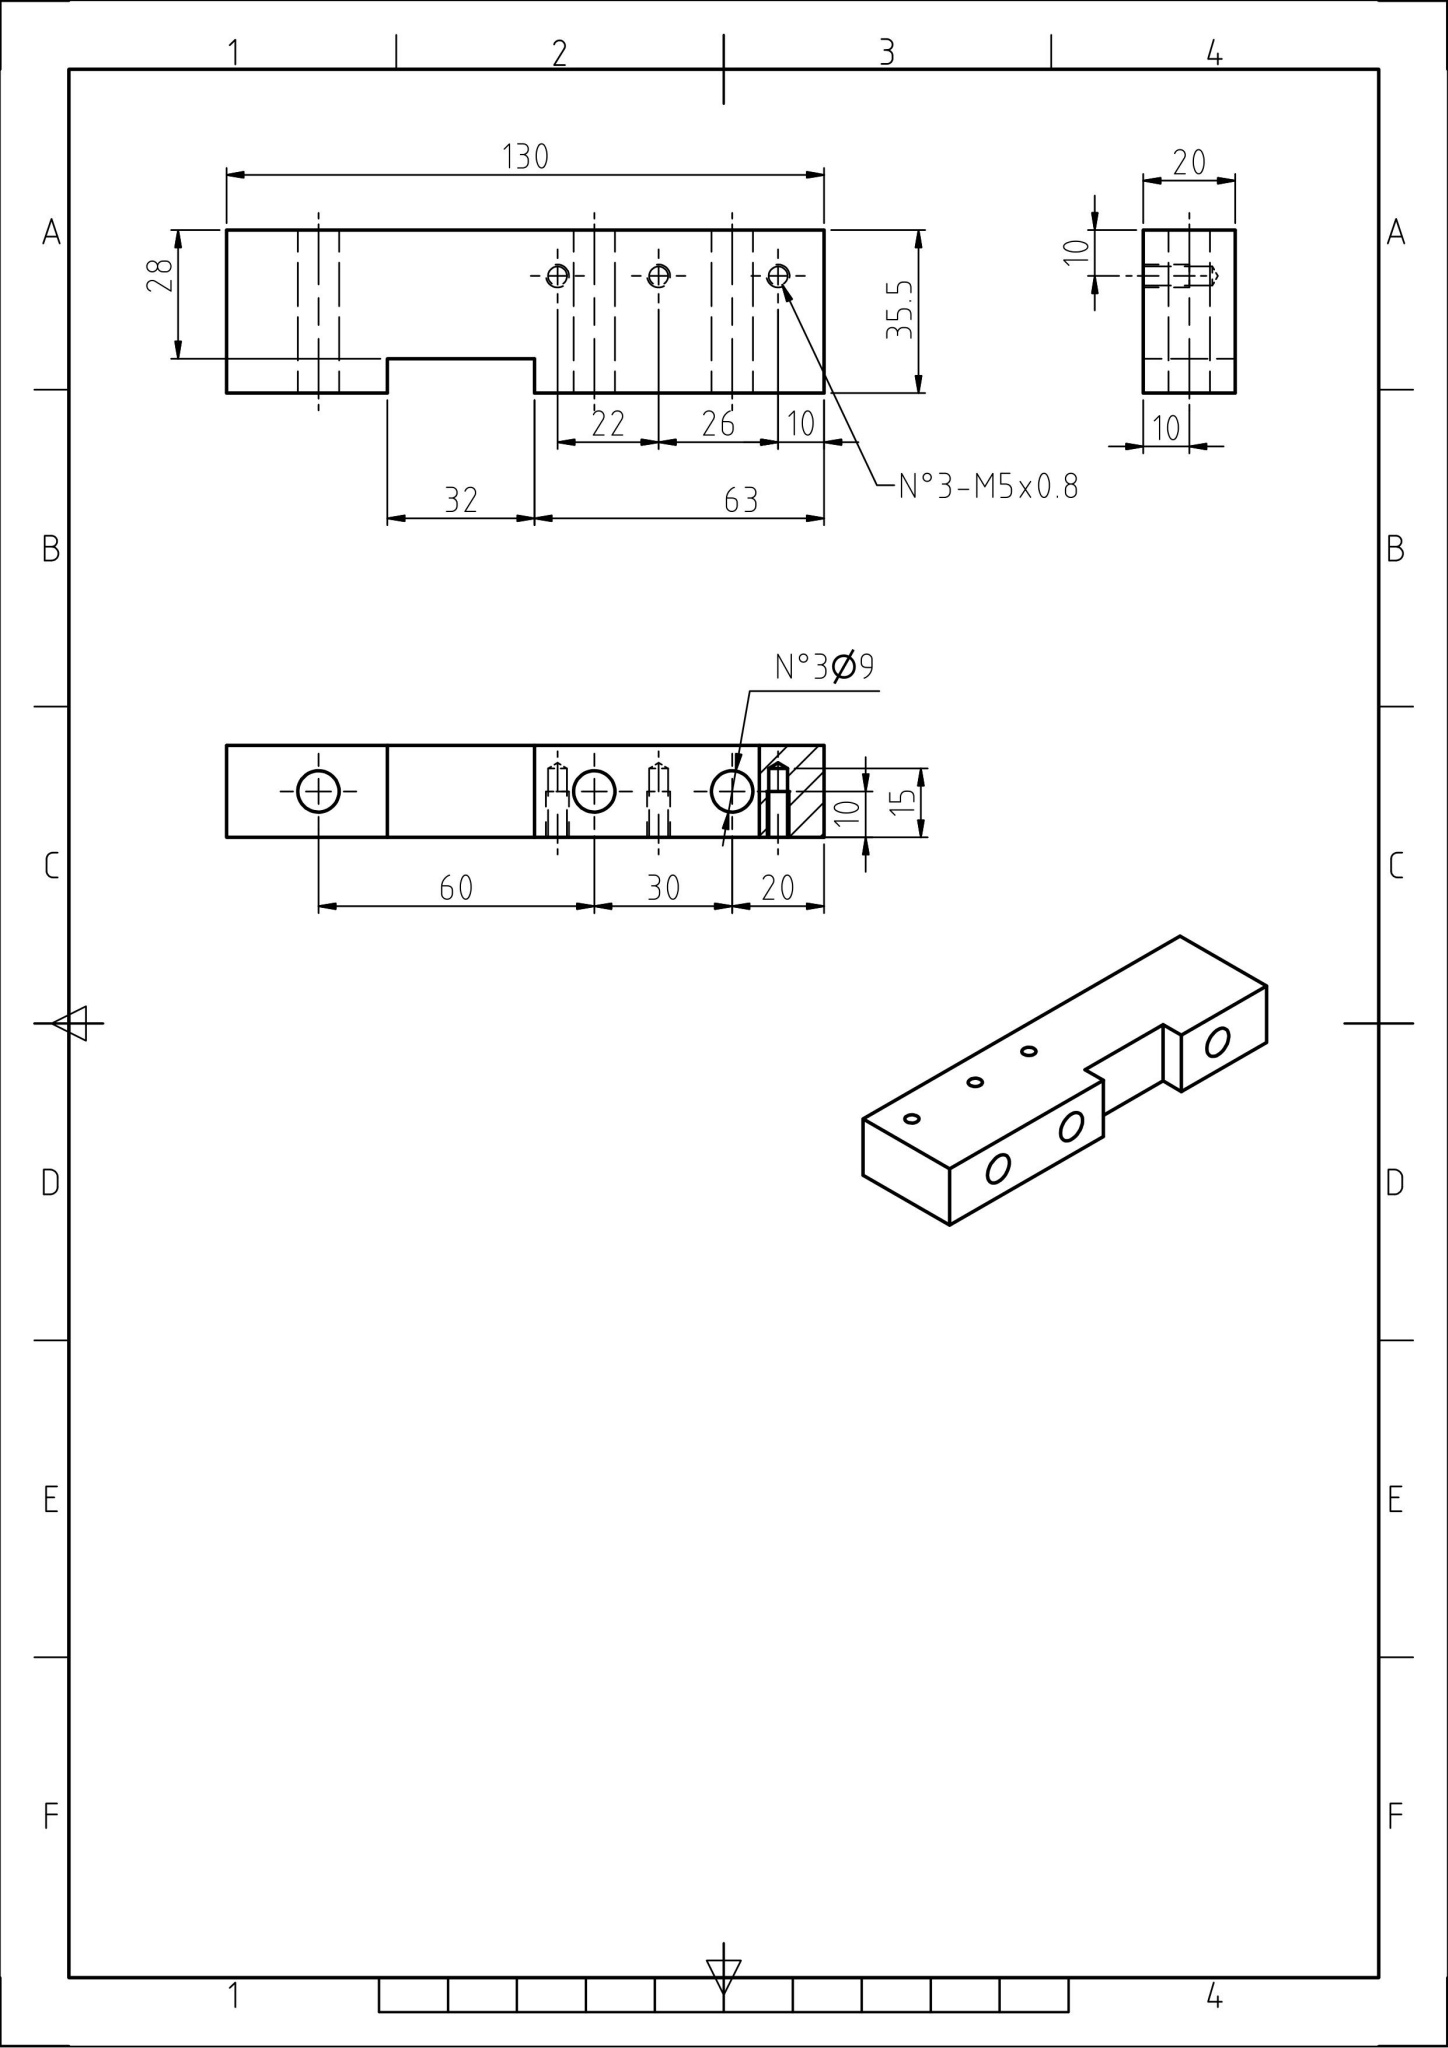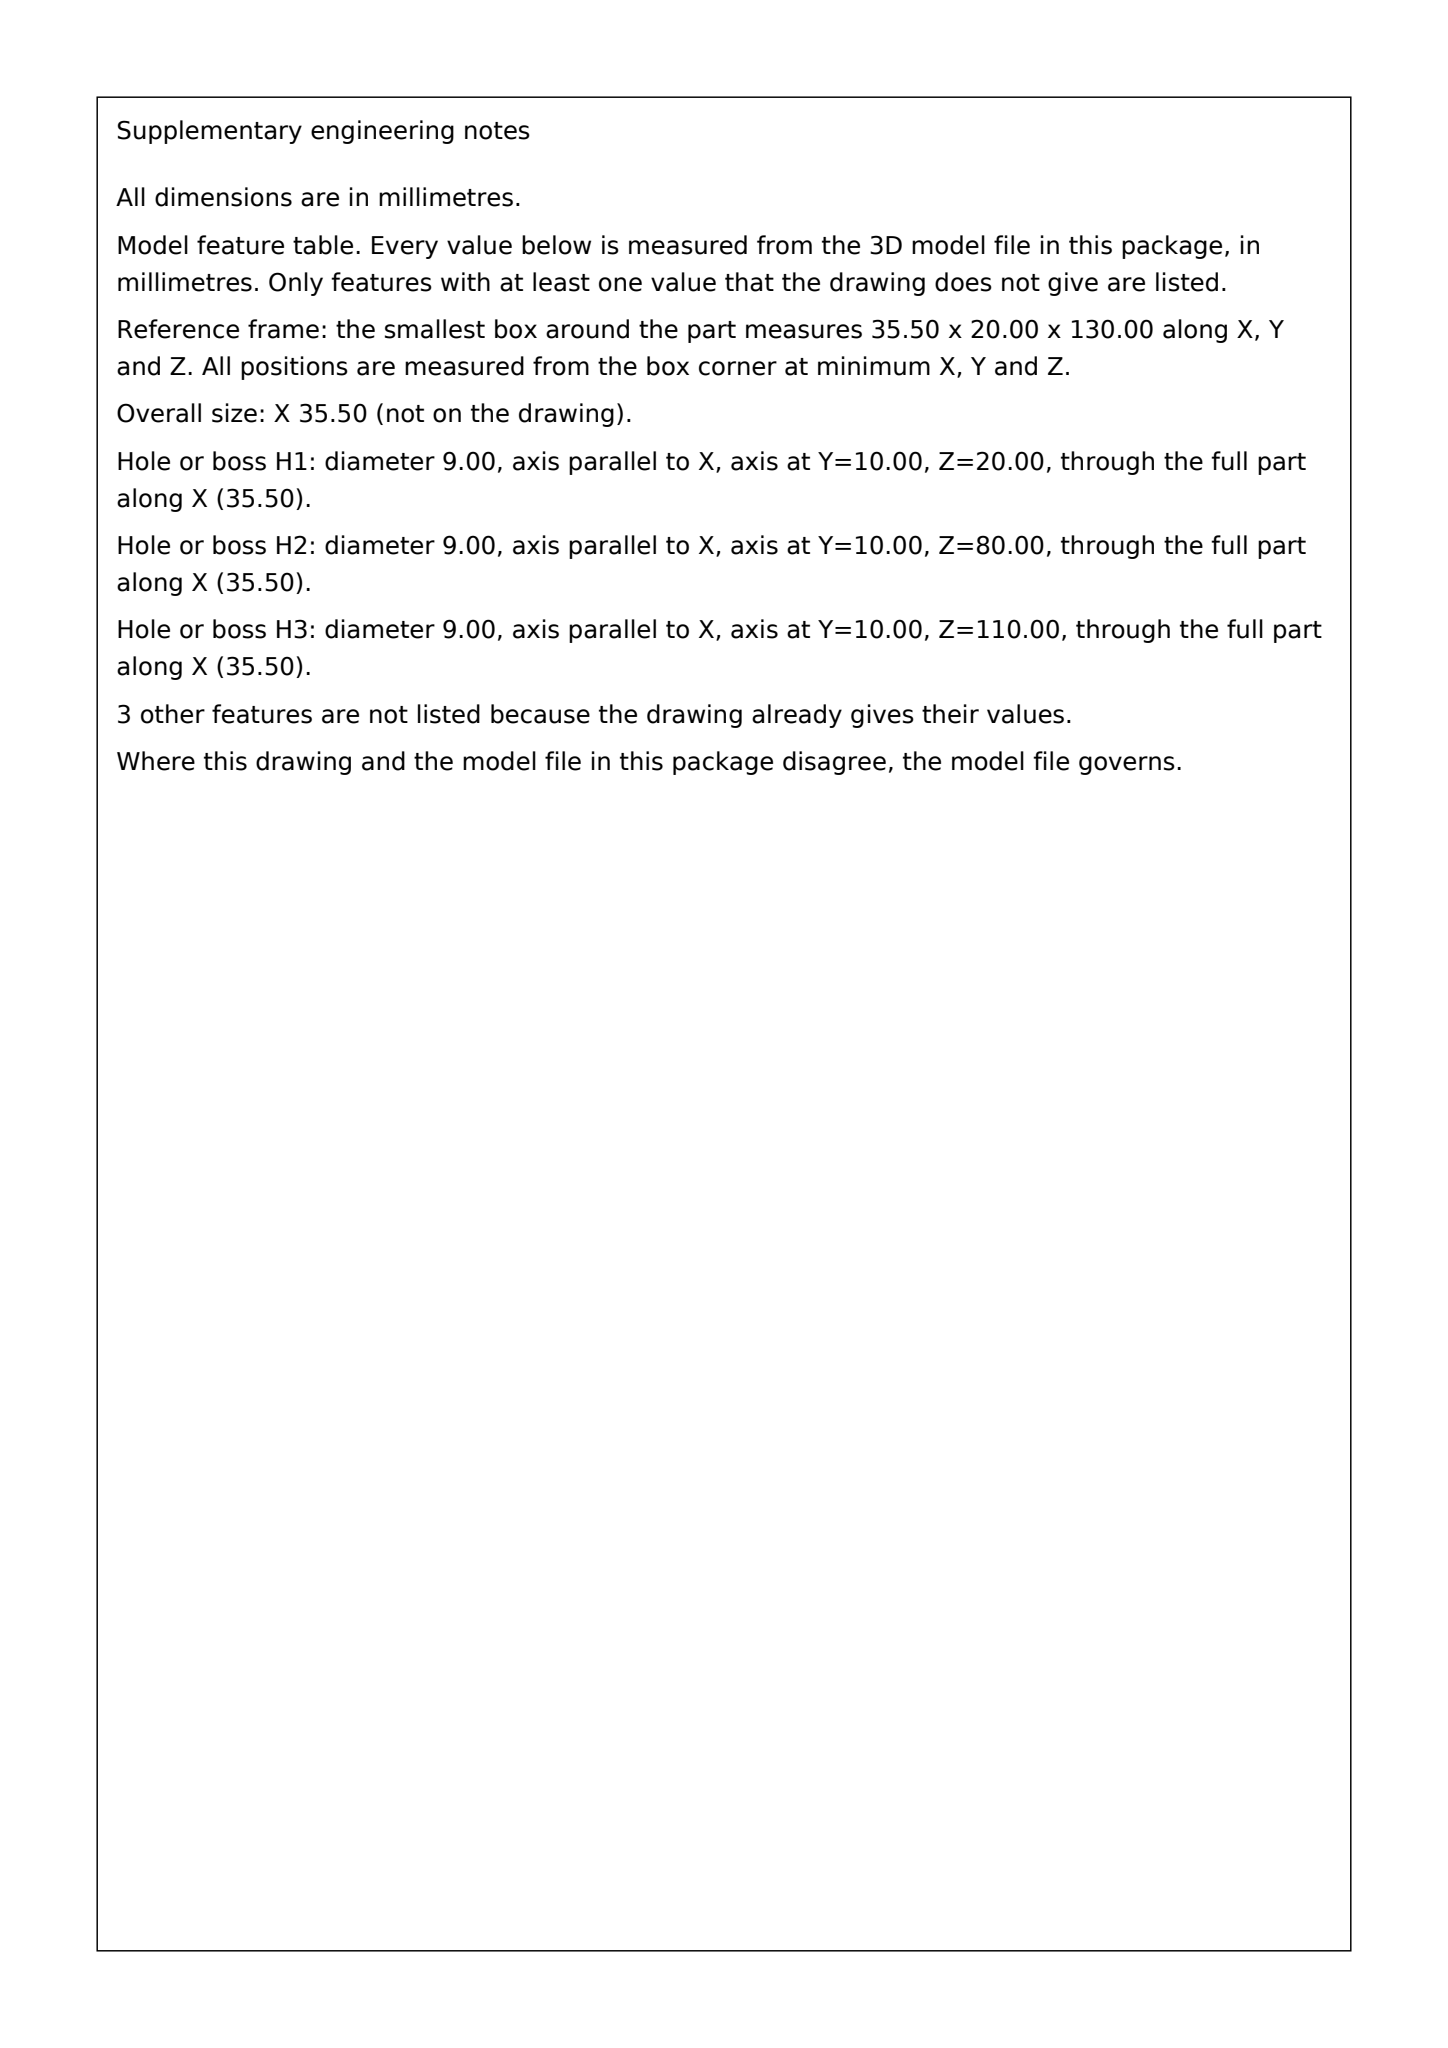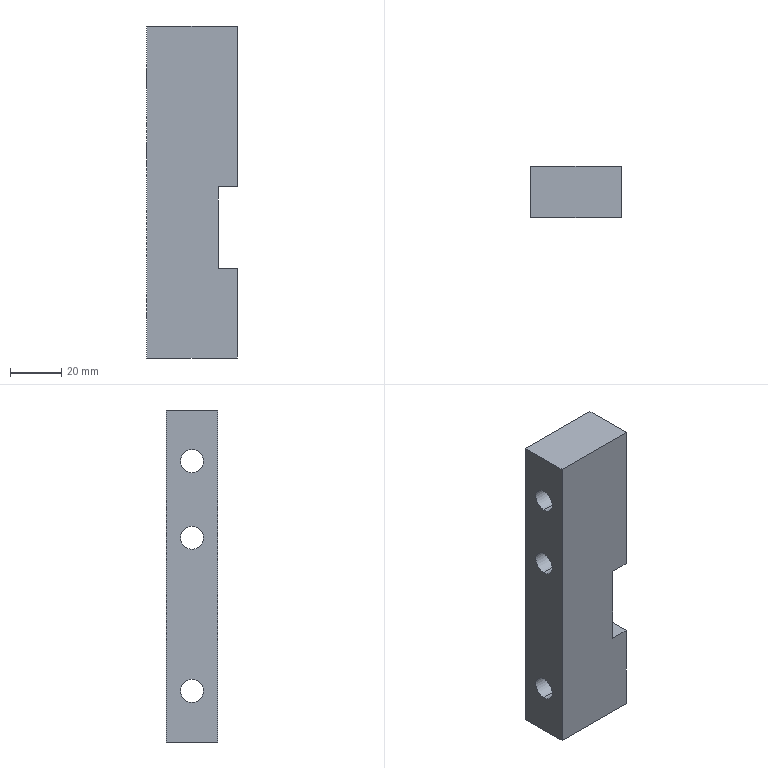Part | SolidWorks | mm | 1 solid | 28 faces | box 35.5 x 20 x 130 mm | volume 80104 mm3 | cylinder 12 | plane 10 | cone 6 | commonest cylinder face diameters 9 x6 4.134 x6
STEP:
#1=CARTESIAN_POINT('',(0.,0.,-40.5));
#2=VERTEX_POINT('',#1);
#3=CARTESIAN_POINT('',(0.,0.,-49.5));
#4=VERTEX_POINT('',#3);
#5=CARTESIAN_POINT('',(0.,0.,-45.));
#6=DIRECTION('',(1.,0.,0.));
#7=DIRECTION('',(0.,0.,-1.));
#8=AXIS2_PLACEMENT_3D('',#5,#6,#7);
#9=CIRCLE('',#8,4.5);
#10=EDGE_CURVE('',#2,#4,#9,.T.);
#11=ORIENTED_EDGE('',*,*,#10,.F.);
#12=CARTESIAN_POINT('',(35.5,0.,-40.5));
#13=VERTEX_POINT('',#12);
#14=CARTESIAN_POINT('',(-100.736,0.,-40.5));
#15=DIRECTION('',(1.,0.,0.));
#16=VECTOR('',#15,1000.);
#17=LINE('',#14,#16);
#18=EDGE_CURVE('',#2,#13,#17,.T.);
#19=ORIENTED_EDGE('',*,*,#18,.T.);
#20=CARTESIAN_POINT('',(35.5,0.,-49.5));
#21=VERTEX_POINT('',#20);
#22=CARTESIAN_POINT('',(35.5,0.,-45.));
#23=DIRECTION('',(-1.,0.,0.));
#24=DIRECTION('',(0.,0.,-1.));
#25=AXIS2_PLACEMENT_3D('',#22,#23,#24);
#26=CIRCLE('',#25,4.5);
#27=EDGE_CURVE('',#21,#13,#26,.T.);
#28=ORIENTED_EDGE('',*,*,#27,.F.);
#29=CARTESIAN_POINT('',(-100.736,0.,-49.5));
#30=DIRECTION('',(1.,0.,0.));
#31=VECTOR('',#30,1000.);
#32=LINE('',#29,#31);
#33=EDGE_CURVE('',#4,#21,#32,.T.);
#34=ORIENTED_EDGE('',*,*,#33,.F.);
#35=EDGE_LOOP('',(#11,#19,#28,#34));
#36=FACE_OUTER_BOUND('',#35,.T.);
#37=CARTESIAN_POINT('',(-100.736,0.,-45.));
#38=DIRECTION('',(1.,0.,0.));
#39=DIRECTION('',(0.,0.,-1.));
#40=AXIS2_PLACEMENT_3D('',#37,#38,#39);
#41=CYLINDRICAL_SURFACE('',#40,4.5);
#42=ADVANCED_FACE('',(#36),#41,.F.);
#43=CARTESIAN_POINT('',(0.,0.,49.5));
#44=VERTEX_POINT('',#43);
#45=CARTESIAN_POINT('',(0.,0.,40.5));
#46=VERTEX_POINT('',#45);
#47=CARTESIAN_POINT('',(0.,0.,45.));
#48=DIRECTION('',(1.,0.,0.));
#49=DIRECTION('',(0.,0.,-1.));
#50=AXIS2_PLACEMENT_3D('',#47,#48,#49);
#51=CIRCLE('',#50,4.5);
#52=EDGE_CURVE('',#44,#46,#51,.T.);
#53=ORIENTED_EDGE('',*,*,#52,.F.);
#54=CARTESIAN_POINT('',(35.5,0.,49.5));
#55=VERTEX_POINT('',#54);
#56=CARTESIAN_POINT('',(-100.736,0.,49.5));
#57=DIRECTION('',(1.,0.,0.));
#58=VECTOR('',#57,1000.);
#59=LINE('',#56,#58);
#60=EDGE_CURVE('',#44,#55,#59,.T.);
#61=ORIENTED_EDGE('',*,*,#60,.T.);
#62=CARTESIAN_POINT('',(35.5,0.,40.5));
#63=VERTEX_POINT('',#62);
#64=CARTESIAN_POINT('',(35.5,0.,45.));
#65=DIRECTION('',(-1.,0.,0.));
#66=DIRECTION('',(0.,0.,-1.));
#67=AXIS2_PLACEMENT_3D('',#64,#65,#66);
#68=CIRCLE('',#67,4.5);
#69=EDGE_CURVE('',#63,#55,#68,.T.);
#70=ORIENTED_EDGE('',*,*,#69,.F.);
#71=CARTESIAN_POINT('',(-100.736,0.,40.5));
#72=DIRECTION('',(1.,0.,0.));
#73=VECTOR('',#72,1000.);
#74=LINE('',#71,#73);
#75=EDGE_CURVE('',#46,#63,#74,.T.);
#76=ORIENTED_EDGE('',*,*,#75,.F.);
#77=EDGE_LOOP('',(#53,#61,#70,#76));
#78=FACE_OUTER_BOUND('',#77,.T.);
#79=CARTESIAN_POINT('',(-100.736,0.,45.));
#80=DIRECTION('',(1.,0.,0.));
#81=DIRECTION('',(0.,0.,-1.));
#82=AXIS2_PLACEMENT_3D('',#79,#80,#81);
#83=CYLINDRICAL_SURFACE('',#82,4.5);
#84=ADVANCED_FACE('',(#78),#83,.F.);
#85=CARTESIAN_POINT('',(0.,0.,19.5));
#86=VERTEX_POINT('',#85);
#87=CARTESIAN_POINT('',(0.,0.,10.5));
#88=VERTEX_POINT('',#87);
#89=CARTESIAN_POINT('',(0.,0.,15.));
#90=DIRECTION('',(1.,0.,0.));
#91=DIRECTION('',(0.,0.,-1.));
#92=AXIS2_PLACEMENT_3D('',#89,#90,#91);
#93=CIRCLE('',#92,4.5);
#94=EDGE_CURVE('',#86,#88,#93,.T.);
#95=ORIENTED_EDGE('',*,*,#94,.F.);
#96=CARTESIAN_POINT('',(35.5,0.,19.5));
#97=VERTEX_POINT('',#96);
#98=CARTESIAN_POINT('',(-100.736,0.,19.5));
#99=DIRECTION('',(1.,0.,0.));
#100=VECTOR('',#99,1000.);
#101=LINE('',#98,#100);
#102=EDGE_CURVE('',#86,#97,#101,.T.);
#103=ORIENTED_EDGE('',*,*,#102,.T.);
#104=CARTESIAN_POINT('',(35.5,0.,10.5));
#105=VERTEX_POINT('',#104);
#106=CARTESIAN_POINT('',(35.5,0.,15.));
#107=DIRECTION('',(-1.,0.,0.));
#108=DIRECTION('',(0.,0.,-1.));
#109=AXIS2_PLACEMENT_3D('',#106,#107,#108);
#110=CIRCLE('',#109,4.5);
#111=EDGE_CURVE('',#105,#97,#110,.T.);
#112=ORIENTED_EDGE('',*,*,#111,.F.);
#113=CARTESIAN_POINT('',(-100.736,0.,10.5));
#114=DIRECTION('',(1.,0.,0.));
#115=VECTOR('',#114,1000.);
#116=LINE('',#113,#115);
#117=EDGE_CURVE('',#88,#105,#116,.T.);
#118=ORIENTED_EDGE('',*,*,#117,.F.);
#119=EDGE_LOOP('',(#95,#103,#112,#118));
#120=FACE_OUTER_BOUND('',#119,.T.);
#121=CARTESIAN_POINT('',(-100.736,0.,15.));
#122=DIRECTION('',(1.,0.,0.));
#123=DIRECTION('',(0.,0.,-1.));
#124=AXIS2_PLACEMENT_3D('',#121,#122,#123);
#125=CYLINDRICAL_SURFACE('',#124,4.5);
#126=ADVANCED_FACE('',(#120),#125,.F.);
#127=CARTESIAN_POINT('',(7.933,-5.,7.));
#128=VERTEX_POINT('',#127);
#129=CARTESIAN_POINT('',(12.067,-5.,7.));
#130=VERTEX_POINT('',#129);
#131=CARTESIAN_POINT('',(10.,-5.,7.));
#132=DIRECTION('',(0.,1.,-0.));
#133=DIRECTION('',(1.,0.,0.));
#134=AXIS2_PLACEMENT_3D('',#131,#132,#133);
#135=CIRCLE('',#134,2.067);
#136=EDGE_CURVE('',#128,#130,#135,.T.);
#137=ORIENTED_EDGE('',*,*,#136,.F.);
#138=CARTESIAN_POINT('',(7.933,10.,7.));
#139=VERTEX_POINT('',#138);
#140=CARTESIAN_POINT('',(7.933,2.5,7.));
#141=DIRECTION('',(0.,1.,-0.));
#142=VECTOR('',#141,1000.);
#143=LINE('',#140,#142);
#144=EDGE_CURVE('',#128,#139,#143,.T.);
#145=ORIENTED_EDGE('',*,*,#144,.T.);
#146=CARTESIAN_POINT('',(12.067,10.,7.));
#147=VERTEX_POINT('',#146);
#148=CARTESIAN_POINT('',(10.,10.,7.));
#149=DIRECTION('',(0.,-1.,0.));
#150=DIRECTION('',(1.,0.,0.));
#151=AXIS2_PLACEMENT_3D('',#148,#149,#150);
#152=CIRCLE('',#151,2.067);
#153=EDGE_CURVE('',#147,#139,#152,.T.);
#154=ORIENTED_EDGE('',*,*,#153,.F.);
#155=CARTESIAN_POINT('',(12.067,2.5,7.));
#156=DIRECTION('',(0.,1.,-0.));
#157=VECTOR('',#156,1000.);
#158=LINE('',#155,#157);
#159=EDGE_CURVE('',#130,#147,#158,.T.);
#160=ORIENTED_EDGE('',*,*,#159,.F.);
#161=EDGE_LOOP('',(#137,#145,#154,#160));
#162=FACE_OUTER_BOUND('',#161,.T.);
#163=CARTESIAN_POINT('',(10.,2.5,7.));
#164=DIRECTION('',(0.,1.,-0.));
#165=DIRECTION('',(1.,0.,0.));
#166=AXIS2_PLACEMENT_3D('',#163,#164,#165);
#167=CYLINDRICAL_SURFACE('',#166,2.067);
#168=ADVANCED_FACE('',(#162),#167,.F.);
#169=CARTESIAN_POINT('',(10.,-6.242,7.));
#170=VERTEX_POINT('',#169);
#171=CARTESIAN_POINT('',(11.034,-5.621,7.));
#172=DIRECTION('',(0.8572,0.515,-0.));
#173=VECTOR('',#172,1000.);
#174=LINE('',#171,#173);
#175=EDGE_CURVE('',#170,#130,#174,.T.);
#176=ORIENTED_EDGE('',*,*,#175,.F.);
#177=CARTESIAN_POINT('',(8.966,-5.621,7.));
#178=DIRECTION('',(-0.8572,0.515,-0.));
#179=VECTOR('',#178,1000.);
#180=LINE('',#177,#179);
#181=EDGE_CURVE('',#170,#128,#180,.T.);
#182=ORIENTED_EDGE('',*,*,#181,.T.);
#183=ORIENTED_EDGE('',*,*,#136,.T.);
#184=EDGE_LOOP('',(#176,#182,#183));
#185=FACE_OUTER_BOUND('',#184,.T.);
#186=CARTESIAN_POINT('',(10.,-5.621,7.));
#187=DIRECTION('',(0.,1.,-0.));
#188=DIRECTION('',(1.,0.,0.));
#189=AXIS2_PLACEMENT_3D('',#186,#187,#188);
#190=CONICAL_SURFACE('',#189,1.033,1.03);
#191=ADVANCED_FACE('',(#185),#190,.F.);
#192=CARTESIAN_POINT('',(7.933,-5.,55.));
#193=VERTEX_POINT('',#192);
#194=CARTESIAN_POINT('',(12.067,-5.,55.));
#195=VERTEX_POINT('',#194);
#196=CARTESIAN_POINT('',(10.,-5.,55.));
#197=DIRECTION('',(0.,1.,-0.));
#198=DIRECTION('',(1.,0.,0.));
#199=AXIS2_PLACEMENT_3D('',#196,#197,#198);
#200=CIRCLE('',#199,2.067);
#201=EDGE_CURVE('',#193,#195,#200,.T.);
#202=ORIENTED_EDGE('',*,*,#201,.F.);
#203=CARTESIAN_POINT('',(7.933,10.,55.));
#204=VERTEX_POINT('',#203);
#205=CARTESIAN_POINT('',(7.933,2.5,55.));
#206=DIRECTION('',(0.,1.,-0.));
#207=VECTOR('',#206,1000.);
#208=LINE('',#205,#207);
#209=EDGE_CURVE('',#193,#204,#208,.T.);
#210=ORIENTED_EDGE('',*,*,#209,.T.);
#211=CARTESIAN_POINT('',(12.067,10.,55.));
#212=VERTEX_POINT('',#211);
#213=CARTESIAN_POINT('',(10.,10.,55.));
#214=DIRECTION('',(0.,-1.,0.));
#215=DIRECTION('',(1.,0.,0.));
#216=AXIS2_PLACEMENT_3D('',#213,#214,#215);
#217=CIRCLE('',#216,2.067);
#218=EDGE_CURVE('',#212,#204,#217,.T.);
#219=ORIENTED_EDGE('',*,*,#218,.F.);
#220=CARTESIAN_POINT('',(12.067,2.5,55.));
#221=DIRECTION('',(0.,1.,-0.));
#222=VECTOR('',#221,1000.);
#223=LINE('',#220,#222);
#224=EDGE_CURVE('',#195,#212,#223,.T.);
#225=ORIENTED_EDGE('',*,*,#224,.F.);
#226=EDGE_LOOP('',(#202,#210,#219,#225));
#227=FACE_OUTER_BOUND('',#226,.T.);
#228=CARTESIAN_POINT('',(10.,2.5,55.));
#229=DIRECTION('',(0.,1.,-0.));
#230=DIRECTION('',(1.,0.,0.));
#231=AXIS2_PLACEMENT_3D('',#228,#229,#230);
#232=CYLINDRICAL_SURFACE('',#231,2.067);
#233=ADVANCED_FACE('',(#227),#232,.F.);
#234=CARTESIAN_POINT('',(10.,-6.242,55.));
#235=VERTEX_POINT('',#234);
#236=CARTESIAN_POINT('',(11.034,-5.621,55.));
#237=DIRECTION('',(0.8572,0.515,-0.));
#238=VECTOR('',#237,1000.);
#239=LINE('',#236,#238);
#240=EDGE_CURVE('',#235,#195,#239,.T.);
#241=ORIENTED_EDGE('',*,*,#240,.F.);
#242=CARTESIAN_POINT('',(8.966,-5.621,55.));
#243=DIRECTION('',(-0.8572,0.515,-0.));
#244=VECTOR('',#243,1000.);
#245=LINE('',#242,#244);
#246=EDGE_CURVE('',#235,#193,#245,.T.);
#247=ORIENTED_EDGE('',*,*,#246,.T.);
#248=ORIENTED_EDGE('',*,*,#201,.T.);
#249=EDGE_LOOP('',(#241,#247,#248));
#250=FACE_OUTER_BOUND('',#249,.T.);
#251=CARTESIAN_POINT('',(10.,-5.621,55.));
#252=DIRECTION('',(0.,1.,-0.));
#253=DIRECTION('',(1.,0.,0.));
#254=AXIS2_PLACEMENT_3D('',#251,#252,#253);
#255=CONICAL_SURFACE('',#254,1.033,1.03);
#256=ADVANCED_FACE('',(#250),#255,.F.);
#257=CARTESIAN_POINT('',(7.933,-5.,29.));
#258=VERTEX_POINT('',#257);
#259=CARTESIAN_POINT('',(12.067,-5.,29.));
#260=VERTEX_POINT('',#259);
#261=CARTESIAN_POINT('',(10.,-5.,29.));
#262=DIRECTION('',(0.,1.,-0.));
#263=DIRECTION('',(1.,0.,0.));
#264=AXIS2_PLACEMENT_3D('',#261,#262,#263);
#265=CIRCLE('',#264,2.067);
#266=EDGE_CURVE('',#258,#260,#265,.T.);
#267=ORIENTED_EDGE('',*,*,#266,.F.);
#268=CARTESIAN_POINT('',(7.933,10.,29.));
#269=VERTEX_POINT('',#268);
#270=CARTESIAN_POINT('',(7.933,2.5,29.));
#271=DIRECTION('',(0.,1.,-0.));
#272=VECTOR('',#271,1000.);
#273=LINE('',#270,#272);
#274=EDGE_CURVE('',#258,#269,#273,.T.);
#275=ORIENTED_EDGE('',*,*,#274,.T.);
#276=CARTESIAN_POINT('',(12.067,10.,29.));
#277=VERTEX_POINT('',#276);
#278=CARTESIAN_POINT('',(10.,10.,29.));
#279=DIRECTION('',(0.,-1.,0.));
#280=DIRECTION('',(1.,0.,0.));
#281=AXIS2_PLACEMENT_3D('',#278,#279,#280);
#282=CIRCLE('',#281,2.067);
#283=EDGE_CURVE('',#277,#269,#282,.T.);
#284=ORIENTED_EDGE('',*,*,#283,.F.);
#285=CARTESIAN_POINT('',(12.067,2.5,29.));
#286=DIRECTION('',(0.,1.,-0.));
#287=VECTOR('',#286,1000.);
#288=LINE('',#285,#287);
#289=EDGE_CURVE('',#260,#277,#288,.T.);
#290=ORIENTED_EDGE('',*,*,#289,.F.);
#291=EDGE_LOOP('',(#267,#275,#284,#290));
#292=FACE_OUTER_BOUND('',#291,.T.);
#293=CARTESIAN_POINT('',(10.,2.5,29.));
#294=DIRECTION('',(0.,1.,-0.));
#295=DIRECTION('',(1.,0.,0.));
#296=AXIS2_PLACEMENT_3D('',#293,#294,#295);
#297=CYLINDRICAL_SURFACE('',#296,2.067);
#298=ADVANCED_FACE('',(#292),#297,.F.);
#299=CARTESIAN_POINT('',(10.,-6.242,29.));
#300=VERTEX_POINT('',#299);
#301=CARTESIAN_POINT('',(11.034,-5.621,29.));
#302=DIRECTION('',(0.8572,0.515,-0.));
#303=VECTOR('',#302,1000.);
#304=LINE('',#301,#303);
#305=EDGE_CURVE('',#300,#260,#304,.T.);
#306=ORIENTED_EDGE('',*,*,#305,.F.);
#307=CARTESIAN_POINT('',(8.966,-5.621,29.));
#308=DIRECTION('',(-0.8572,0.515,-0.));
#309=VECTOR('',#308,1000.);
#310=LINE('',#307,#309);
#311=EDGE_CURVE('',#300,#258,#310,.T.);
#312=ORIENTED_EDGE('',*,*,#311,.T.);
#313=ORIENTED_EDGE('',*,*,#266,.T.);
#314=EDGE_LOOP('',(#306,#312,#313));
#315=FACE_OUTER_BOUND('',#314,.T.);
#316=CARTESIAN_POINT('',(10.,-5.621,29.));
#317=DIRECTION('',(0.,1.,-0.));
#318=DIRECTION('',(1.,0.,0.));
#319=AXIS2_PLACEMENT_3D('',#316,#317,#318);
#320=CONICAL_SURFACE('',#319,1.033,1.03);
#321=ADVANCED_FACE('',(#315),#320,.F.);
#322=CARTESIAN_POINT('',(28.,-10.,2.));
#323=VERTEX_POINT('',#322);
#324=CARTESIAN_POINT('',(35.5,-10.,2.));
#325=VERTEX_POINT('',#324);
#326=CARTESIAN_POINT('',(24.,-10.,2.));
#327=DIRECTION('',(1.,0.,0.));
#328=VECTOR('',#327,1000.);
#329=LINE('',#326,#328);
#330=EDGE_CURVE('',#323,#325,#329,.T.);
#331=ORIENTED_EDGE('',*,*,#330,.F.);
#332=CARTESIAN_POINT('',(28.,10.,2.));
#333=VERTEX_POINT('',#332);
#334=CARTESIAN_POINT('',(28.,10.,2.));
#335=DIRECTION('',(0.,-1.,0.));
#336=VECTOR('',#335,1000.);
#337=LINE('',#334,#336);
#338=EDGE_CURVE('',#333,#323,#337,.T.);
#339=ORIENTED_EDGE('',*,*,#338,.F.);
#340=CARTESIAN_POINT('',(35.5,10.,2.));
#341=VERTEX_POINT('',#340);
#342=CARTESIAN_POINT('',(24.,10.,2.));
#343=DIRECTION('',(-1.,0.,0.));
#344=VECTOR('',#343,1000.);
#345=LINE('',#342,#344);
#346=EDGE_CURVE('',#341,#333,#345,.T.);
#347=ORIENTED_EDGE('',*,*,#346,.F.);
#348=CARTESIAN_POINT('',(35.5,5.,2.));
#349=DIRECTION('',(0.,1.,-0.));
#350=VECTOR('',#349,1000.);
#351=LINE('',#348,#350);
#352=EDGE_CURVE('',#325,#341,#351,.T.);
#353=ORIENTED_EDGE('',*,*,#352,.F.);
#354=EDGE_LOOP('',(#331,#339,#347,#353));
#355=FACE_OUTER_BOUND('',#354,.T.);
#356=CARTESIAN_POINT('',(48.,10.,2.));
#357=DIRECTION('',(0.,0.,1.));
#358=DIRECTION('',(1.,0.,0.));
#359=AXIS2_PLACEMENT_3D('',#356,#357,#358);
#360=PLANE('',#359);
#361=ADVANCED_FACE('',(#355),#360,.F.);
#362=CARTESIAN_POINT('',(35.5,-10.,-30.));
#363=VERTEX_POINT('',#362);
#364=CARTESIAN_POINT('',(28.,-10.,-30.));
#365=VERTEX_POINT('',#364);
#366=CARTESIAN_POINT('',(14.,-10.,-30.));
#367=DIRECTION('',(-1.,0.,0.));
#368=VECTOR('',#367,1000.);
#369=LINE('',#366,#368);
#370=EDGE_CURVE('',#363,#365,#369,.T.);
#371=ORIENTED_EDGE('',*,*,#370,.F.);
#372=CARTESIAN_POINT('',(35.5,10.,-30.));
#373=VERTEX_POINT('',#372);
#374=CARTESIAN_POINT('',(35.5,5.,-30.));
#375=DIRECTION('',(0.,-1.,0.));
#376=VECTOR('',#375,1000.);
#377=LINE('',#374,#376);
#378=EDGE_CURVE('',#373,#363,#377,.T.);
#379=ORIENTED_EDGE('',*,*,#378,.F.);
#380=CARTESIAN_POINT('',(28.,10.,-30.));
#381=VERTEX_POINT('',#380);
#382=CARTESIAN_POINT('',(14.,10.,-30.));
#383=DIRECTION('',(1.,0.,0.));
#384=VECTOR('',#383,1000.);
#385=LINE('',#382,#384);
#386=EDGE_CURVE('',#381,#373,#385,.T.);
#387=ORIENTED_EDGE('',*,*,#386,.F.);
#388=CARTESIAN_POINT('',(28.,10.,-30.));
#389=DIRECTION('',(0.,-1.,0.));
#390=VECTOR('',#389,1000.);
#391=LINE('',#388,#390);
#392=EDGE_CURVE('',#381,#365,#391,.T.);
#393=ORIENTED_EDGE('',*,*,#392,.T.);
#394=EDGE_LOOP('',(#371,#379,#387,#393));
#395=FACE_OUTER_BOUND('',#394,.T.);
#396=CARTESIAN_POINT('',(28.,10.,-30.));
#397=DIRECTION('',(0.,-0.,-1.));
#398=DIRECTION('',(0.,-1.,0.));
#399=AXIS2_PLACEMENT_3D('',#396,#397,#398);
#400=PLANE('',#399);
#401=ADVANCED_FACE('',(#395),#400,.F.);
#402=CARTESIAN_POINT('',(28.,-10.,33.5));
#403=DIRECTION('',(0.,-0.,1.));
#404=VECTOR('',#403,1000.);
#405=LINE('',#402,#404);
#406=EDGE_CURVE('',#365,#323,#405,.T.);
#407=ORIENTED_EDGE('',*,*,#406,.F.);
#408=ORIENTED_EDGE('',*,*,#392,.F.);
#409=CARTESIAN_POINT('',(28.,10.,-31.5));
#410=DIRECTION('',(-0.,-0.,-1.));
#411=VECTOR('',#410,1000.);
#412=LINE('',#409,#411);
#413=EDGE_CURVE('',#333,#381,#412,.T.);
#414=ORIENTED_EDGE('',*,*,#413,.F.);
#415=ORIENTED_EDGE('',*,*,#338,.T.);
#416=EDGE_LOOP('',(#407,#408,#414,#415));
#417=FACE_OUTER_BOUND('',#416,.T.);
#418=CARTESIAN_POINT('',(28.,10.,2.));
#419=DIRECTION('',(-1.,0.,0.));
#420=DIRECTION('',(0.,1.,0.));
#421=AXIS2_PLACEMENT_3D('',#418,#419,#420);
#422=PLANE('',#421);
#423=ADVANCED_FACE('',(#417),#422,.F.);
#424=ORIENTED_EDGE('',*,*,#378,.T.);
#425=CARTESIAN_POINT('',(35.5,-10.,-65.));
#426=VERTEX_POINT('',#425);
#427=CARTESIAN_POINT('',(35.5,-10.,65.));
#428=DIRECTION('',(0.,0.,-1.));
#429=VECTOR('',#428,1000.);
#430=LINE('',#427,#429);
#431=EDGE_CURVE('',#363,#426,#430,.T.);
#432=ORIENTED_EDGE('',*,*,#431,.T.);
#433=CARTESIAN_POINT('',(35.5,10.,-65.));
#434=VERTEX_POINT('',#433);
#435=CARTESIAN_POINT('',(35.5,-10.,-65.));
#436=DIRECTION('',(0.,1.,0.));
#437=VECTOR('',#436,1000.);
#438=LINE('',#435,#437);
#439=EDGE_CURVE('',#426,#434,#438,.T.);
#440=ORIENTED_EDGE('',*,*,#439,.T.);
#441=CARTESIAN_POINT('',(35.5,10.,-65.));
#442=DIRECTION('',(0.,0.,1.));
#443=VECTOR('',#442,1000.);
#444=LINE('',#441,#443);
#445=EDGE_CURVE('',#434,#373,#444,.T.);
#446=ORIENTED_EDGE('',*,*,#445,.T.);
#447=EDGE_LOOP('',(#424,#432,#440,#446));
#448=FACE_OUTER_BOUND('',#447,.T.);
#449=ORIENTED_EDGE('',*,*,#27,.T.);
#450=CARTESIAN_POINT('',(35.5,0.,-45.));
#451=DIRECTION('',(-1.,0.,0.));
#452=DIRECTION('',(0.,0.,-1.));
#453=AXIS2_PLACEMENT_3D('',#450,#451,#452);
#454=CIRCLE('',#453,4.5);
#455=EDGE_CURVE('',#13,#21,#454,.T.);
#456=ORIENTED_EDGE('',*,*,#455,.T.);
#457=EDGE_LOOP('',(#449,#456));
#458=FACE_BOUND('',#457,.T.);
#459=CARTESIAN_POINT('',(35.5,0.,0.));
#460=DIRECTION('',(1.,0.,0.));
#461=DIRECTION('',(0.,1.,0.));
#462=AXIS2_PLACEMENT_3D('',#459,#460,#461);
#463=PLANE('',#462);
#464=ADVANCED_FACE('',(#448,#458),#463,.T.);
#465=ORIENTED_EDGE('',*,*,#352,.T.);
#466=CARTESIAN_POINT('',(35.5,10.,65.));
#467=VERTEX_POINT('',#466);
#468=CARTESIAN_POINT('',(35.5,10.,-65.));
#469=DIRECTION('',(0.,0.,1.));
#470=VECTOR('',#469,1000.);
#471=LINE('',#468,#470);
#472=EDGE_CURVE('',#341,#467,#471,.T.);
#473=ORIENTED_EDGE('',*,*,#472,.T.);
#474=CARTESIAN_POINT('',(35.5,-10.,65.));
#475=VERTEX_POINT('',#474);
#476=CARTESIAN_POINT('',(35.5,10.,65.));
#477=DIRECTION('',(0.,-1.,0.));
#478=VECTOR('',#477,1000.);
#479=LINE('',#476,#478);
#480=EDGE_CURVE('',#467,#475,#479,.T.);
#481=ORIENTED_EDGE('',*,*,#480,.T.);
#482=CARTESIAN_POINT('',(35.5,-10.,65.));
#483=DIRECTION('',(0.,0.,-1.));
#484=VECTOR('',#483,1000.);
#485=LINE('',#482,#484);
#486=EDGE_CURVE('',#475,#325,#485,.T.);
#487=ORIENTED_EDGE('',*,*,#486,.T.);
#488=EDGE_LOOP('',(#465,#473,#481,#487));
#489=FACE_OUTER_BOUND('',#488,.T.);
#490=ORIENTED_EDGE('',*,*,#69,.T.);
#491=CARTESIAN_POINT('',(35.5,0.,45.));
#492=DIRECTION('',(-1.,0.,0.));
#493=DIRECTION('',(0.,0.,-1.));
#494=AXIS2_PLACEMENT_3D('',#491,#492,#493);
#495=CIRCLE('',#494,4.5);
#496=EDGE_CURVE('',#55,#63,#495,.T.);
#497=ORIENTED_EDGE('',*,*,#496,.T.);
#498=EDGE_LOOP('',(#490,#497));
#499=FACE_BOUND('',#498,.T.);
#500=ORIENTED_EDGE('',*,*,#111,.T.);
#501=CARTESIAN_POINT('',(35.5,0.,15.));
#502=DIRECTION('',(-1.,0.,0.));
#503=DIRECTION('',(0.,0.,-1.));
#504=AXIS2_PLACEMENT_3D('',#501,#502,#503);
#505=CIRCLE('',#504,4.5);
#506=EDGE_CURVE('',#97,#105,#505,.T.);
#507=ORIENTED_EDGE('',*,*,#506,.T.);
#508=EDGE_LOOP('',(#500,#507));
#509=FACE_BOUND('',#508,.T.);
#510=CARTESIAN_POINT('',(35.5,0.,0.));
#511=DIRECTION('',(1.,0.,0.));
#512=DIRECTION('',(0.,1.,0.));
#513=AXIS2_PLACEMENT_3D('',#510,#511,#512);
#514=PLANE('',#513);
#515=ADVANCED_FACE('',(#489,#499,#509),#514,.T.);
#516=ORIENTED_EDGE('',*,*,#346,.T.);
#517=ORIENTED_EDGE('',*,*,#413,.T.);
#518=ORIENTED_EDGE('',*,*,#386,.T.);
#519=ORIENTED_EDGE('',*,*,#445,.F.);
#520=CARTESIAN_POINT('',(0.,10.,-65.));
#521=VERTEX_POINT('',#520);
#522=CARTESIAN_POINT('',(0.,10.,-65.));
#523=DIRECTION('',(1.,0.,0.));
#524=VECTOR('',#523,1000.);
#525=LINE('',#522,#524);
#526=EDGE_CURVE('',#521,#434,#525,.T.);
#527=ORIENTED_EDGE('',*,*,#526,.F.);
#528=CARTESIAN_POINT('',(0.,10.,65.));
#529=VERTEX_POINT('',#528);
#530=CARTESIAN_POINT('',(0.,10.,-65.));
#531=DIRECTION('',(0.,0.,1.));
#532=VECTOR('',#531,1000.);
#533=LINE('',#530,#532);
#534=EDGE_CURVE('',#521,#529,#533,.T.);
#535=ORIENTED_EDGE('',*,*,#534,.T.);
#536=CARTESIAN_POINT('',(0.,10.,65.));
#537=DIRECTION('',(1.,0.,0.));
#538=VECTOR('',#537,1000.);
#539=LINE('',#536,#538);
#540=EDGE_CURVE('',#529,#467,#539,.T.);
#541=ORIENTED_EDGE('',*,*,#540,.T.);
#542=ORIENTED_EDGE('',*,*,#472,.F.);
#543=EDGE_LOOP('',(#516,#517,#518,#519,#527,#535,#541,#542));
#544=FACE_OUTER_BOUND('',#543,.T.);
#545=ORIENTED_EDGE('',*,*,#153,.T.);
#546=CARTESIAN_POINT('',(10.,10.,7.));
#547=DIRECTION('',(0.,-1.,0.));
#548=DIRECTION('',(1.,0.,0.));
#549=AXIS2_PLACEMENT_3D('',#546,#547,#548);
#550=CIRCLE('',#549,2.067);
#551=EDGE_CURVE('',#139,#147,#550,.T.);
#552=ORIENTED_EDGE('',*,*,#551,.T.);
#553=EDGE_LOOP('',(#545,#552));
#554=FACE_BOUND('',#553,.T.);
#555=ORIENTED_EDGE('',*,*,#218,.T.);
#556=CARTESIAN_POINT('',(10.,10.,55.));
#557=DIRECTION('',(0.,-1.,0.));
#558=DIRECTION('',(1.,0.,0.));
#559=AXIS2_PLACEMENT_3D('',#556,#557,#558);
#560=CIRCLE('',#559,2.067);
#561=EDGE_CURVE('',#204,#212,#560,.T.);
#562=ORIENTED_EDGE('',*,*,#561,.T.);
#563=EDGE_LOOP('',(#555,#562));
#564=FACE_BOUND('',#563,.T.);
#565=ORIENTED_EDGE('',*,*,#283,.T.);
#566=CARTESIAN_POINT('',(10.,10.,29.));
#567=DIRECTION('',(0.,-1.,0.));
#568=DIRECTION('',(1.,0.,0.));
#569=AXIS2_PLACEMENT_3D('',#566,#567,#568);
#570=CIRCLE('',#569,2.067);
#571=EDGE_CURVE('',#269,#277,#570,.T.);
#572=ORIENTED_EDGE('',*,*,#571,.T.);
#573=EDGE_LOOP('',(#565,#572));
#574=FACE_BOUND('',#573,.T.);
#575=CARTESIAN_POINT('',(0.,10.,-65.));
#576=DIRECTION('',(0.,1.,-0.));
#577=DIRECTION('',(1.,0.,0.));
#578=AXIS2_PLACEMENT_3D('',#575,#576,#577);
#579=PLANE('',#578);
#580=ADVANCED_FACE('',(#544,#554,#564,#574),#579,.T.);
#581=ORIENTED_EDGE('',*,*,#311,.F.);
#582=ORIENTED_EDGE('',*,*,#305,.T.);
#583=CARTESIAN_POINT('',(10.,-5.,29.));
#584=DIRECTION('',(0.,1.,-0.));
#585=DIRECTION('',(1.,0.,0.));
#586=AXIS2_PLACEMENT_3D('',#583,#584,#585);
#587=CIRCLE('',#586,2.067);
#588=EDGE_CURVE('',#260,#258,#587,.T.);
#589=ORIENTED_EDGE('',*,*,#588,.T.);
#590=EDGE_LOOP('',(#581,#582,#589));
#591=FACE_OUTER_BOUND('',#590,.T.);
#592=CARTESIAN_POINT('',(10.,-5.621,29.));
#593=DIRECTION('',(0.,1.,-0.));
#594=DIRECTION('',(1.,0.,0.));
#595=AXIS2_PLACEMENT_3D('',#592,#593,#594);
#596=CONICAL_SURFACE('',#595,1.033,1.03);
#597=ADVANCED_FACE('',(#591),#596,.F.);
#598=ORIENTED_EDGE('',*,*,#274,.F.);
#599=ORIENTED_EDGE('',*,*,#588,.F.);
#600=ORIENTED_EDGE('',*,*,#289,.T.);
#601=ORIENTED_EDGE('',*,*,#571,.F.);
#602=EDGE_LOOP('',(#598,#599,#600,#601));
#603=FACE_OUTER_BOUND('',#602,.T.);
#604=CARTESIAN_POINT('',(10.,2.5,29.));
#605=DIRECTION('',(0.,1.,-0.));
#606=DIRECTION('',(1.,0.,0.));
#607=AXIS2_PLACEMENT_3D('',#604,#605,#606);
#608=CYLINDRICAL_SURFACE('',#607,2.067);
#609=ADVANCED_FACE('',(#603),#608,.F.);
#610=ORIENTED_EDGE('',*,*,#246,.F.);
#611=ORIENTED_EDGE('',*,*,#240,.T.);
#612=CARTESIAN_POINT('',(10.,-5.,55.));
#613=DIRECTION('',(0.,1.,-0.));
#614=DIRECTION('',(1.,0.,0.));
#615=AXIS2_PLACEMENT_3D('',#612,#613,#614);
#616=CIRCLE('',#615,2.067);
#617=EDGE_CURVE('',#195,#193,#616,.T.);
#618=ORIENTED_EDGE('',*,*,#617,.T.);
#619=EDGE_LOOP('',(#610,#611,#618));
#620=FACE_OUTER_BOUND('',#619,.T.);
#621=CARTESIAN_POINT('',(10.,-5.621,55.));
#622=DIRECTION('',(0.,1.,-0.));
#623=DIRECTION('',(1.,0.,0.));
#624=AXIS2_PLACEMENT_3D('',#621,#622,#623);
#625=CONICAL_SURFACE('',#624,1.033,1.03);
#626=ADVANCED_FACE('',(#620),#625,.F.);
#627=ORIENTED_EDGE('',*,*,#209,.F.);
#628=ORIENTED_EDGE('',*,*,#617,.F.);
#629=ORIENTED_EDGE('',*,*,#224,.T.);
#630=ORIENTED_EDGE('',*,*,#561,.F.);
#631=EDGE_LOOP('',(#627,#628,#629,#630));
#632=FACE_OUTER_BOUND('',#631,.T.);
#633=CARTESIAN_POINT('',(10.,2.5,55.));
#634=DIRECTION('',(0.,1.,-0.));
#635=DIRECTION('',(1.,0.,0.));
#636=AXIS2_PLACEMENT_3D('',#633,#634,#635);
#637=CYLINDRICAL_SURFACE('',#636,2.067);
#638=ADVANCED_FACE('',(#632),#637,.F.);
#639=ORIENTED_EDGE('',*,*,#181,.F.);
#640=ORIENTED_EDGE('',*,*,#175,.T.);
#641=CARTESIAN_POINT('',(10.,-5.,7.));
#642=DIRECTION('',(0.,1.,-0.));
#643=DIRECTION('',(1.,0.,0.));
#644=AXIS2_PLACEMENT_3D('',#641,#642,#643);
#645=CIRCLE('',#644,2.067);
#646=EDGE_CURVE('',#130,#128,#645,.T.);
#647=ORIENTED_EDGE('',*,*,#646,.T.);
#648=EDGE_LOOP('',(#639,#640,#647));
#649=FACE_OUTER_BOUND('',#648,.T.);
#650=CARTESIAN_POINT('',(10.,-5.621,7.));
#651=DIRECTION('',(0.,1.,-0.));
#652=DIRECTION('',(1.,0.,0.));
#653=AXIS2_PLACEMENT_3D('',#650,#651,#652);
#654=CONICAL_SURFACE('',#653,1.033,1.03);
#655=ADVANCED_FACE('',(#649),#654,.F.);
#656=ORIENTED_EDGE('',*,*,#144,.F.);
#657=ORIENTED_EDGE('',*,*,#646,.F.);
#658=ORIENTED_EDGE('',*,*,#159,.T.);
#659=ORIENTED_EDGE('',*,*,#551,.F.);
#660=EDGE_LOOP('',(#656,#657,#658,#659));
#661=FACE_OUTER_BOUND('',#660,.T.);
#662=CARTESIAN_POINT('',(10.,2.5,7.));
#663=DIRECTION('',(0.,1.,-0.));
#664=DIRECTION('',(1.,0.,0.));
#665=AXIS2_PLACEMENT_3D('',#662,#663,#664);
#666=CYLINDRICAL_SURFACE('',#665,2.067);
#667=ADVANCED_FACE('',(#661),#666,.F.);
#668=ORIENTED_EDGE('',*,*,#102,.F.);
#669=CARTESIAN_POINT('',(0.,0.,15.));
#670=DIRECTION('',(1.,0.,0.));
#671=DIRECTION('',(0.,0.,-1.));
#672=AXIS2_PLACEMENT_3D('',#669,#670,#671);
#673=CIRCLE('',#672,4.5);
#674=EDGE_CURVE('',#88,#86,#673,.T.);
#675=ORIENTED_EDGE('',*,*,#674,.F.);
#676=ORIENTED_EDGE('',*,*,#117,.T.);
#677=ORIENTED_EDGE('',*,*,#506,.F.);
#678=EDGE_LOOP('',(#668,#675,#676,#677));
#679=FACE_OUTER_BOUND('',#678,.T.);
#680=CARTESIAN_POINT('',(-100.736,0.,15.));
#681=DIRECTION('',(1.,0.,0.));
#682=DIRECTION('',(0.,0.,-1.));
#683=AXIS2_PLACEMENT_3D('',#680,#681,#682);
#684=CYLINDRICAL_SURFACE('',#683,4.5);
#685=ADVANCED_FACE('',(#679),#684,.F.);
#686=ORIENTED_EDGE('',*,*,#60,.F.);
#687=CARTESIAN_POINT('',(0.,0.,45.));
#688=DIRECTION('',(1.,0.,0.));
#689=DIRECTION('',(0.,0.,-1.));
#690=AXIS2_PLACEMENT_3D('',#687,#688,#689);
#691=CIRCLE('',#690,4.5);
#692=EDGE_CURVE('',#46,#44,#691,.T.);
#693=ORIENTED_EDGE('',*,*,#692,.F.);
#694=ORIENTED_EDGE('',*,*,#75,.T.);
#695=ORIENTED_EDGE('',*,*,#496,.F.);
#696=EDGE_LOOP('',(#686,#693,#694,#695));
#697=FACE_OUTER_BOUND('',#696,.T.);
#698=CARTESIAN_POINT('',(-100.736,0.,45.));
#699=DIRECTION('',(1.,0.,0.));
#700=DIRECTION('',(0.,0.,-1.));
#701=AXIS2_PLACEMENT_3D('',#698,#699,#700);
#702=CYLINDRICAL_SURFACE('',#701,4.5);
#703=ADVANCED_FACE('',(#697),#702,.F.);
#704=ORIENTED_EDGE('',*,*,#18,.F.);
#705=CARTESIAN_POINT('',(0.,0.,-45.));
#706=DIRECTION('',(1.,0.,0.));
#707=DIRECTION('',(0.,0.,-1.));
#708=AXIS2_PLACEMENT_3D('',#705,#706,#707);
#709=CIRCLE('',#708,4.5);
#710=EDGE_CURVE('',#4,#2,#709,.T.);
#711=ORIENTED_EDGE('',*,*,#710,.F.);
#712=ORIENTED_EDGE('',*,*,#33,.T.);
#713=ORIENTED_EDGE('',*,*,#455,.F.);
#714=EDGE_LOOP('',(#704,#711,#712,#713));
#715=FACE_OUTER_BOUND('',#714,.T.);
#716=CARTESIAN_POINT('',(-100.736,0.,-45.));
#717=DIRECTION('',(1.,0.,0.));
#718=DIRECTION('',(0.,0.,-1.));
#719=AXIS2_PLACEMENT_3D('',#716,#717,#718);
#720=CYLINDRICAL_SURFACE('',#719,4.5);
#721=ADVANCED_FACE('',(#715),#720,.F.);
#722=CARTESIAN_POINT('',(0.,-10.,-65.));
#723=VERTEX_POINT('',#722);
#724=CARTESIAN_POINT('',(0.,-10.,-65.));
#725=DIRECTION('',(0.,1.,0.));
#726=VECTOR('',#725,1000.);
#727=LINE('',#724,#726);
#728=EDGE_CURVE('',#723,#521,#727,.T.);
#729=ORIENTED_EDGE('',*,*,#728,.T.);
#730=ORIENTED_EDGE('',*,*,#526,.T.);
#731=ORIENTED_EDGE('',*,*,#439,.F.);
#732=CARTESIAN_POINT('',(0.,-10.,-65.));
#733=DIRECTION('',(1.,0.,0.));
#734=VECTOR('',#733,1000.);
#735=LINE('',#732,#734);
#736=EDGE_CURVE('',#723,#426,#735,.T.);
#737=ORIENTED_EDGE('',*,*,#736,.F.);
#738=EDGE_LOOP('',(#729,#730,#731,#737));
#739=FACE_OUTER_BOUND('',#738,.T.);
#740=CARTESIAN_POINT('',(0.,-10.,-65.));
#741=DIRECTION('',(0.,0.,-1.));
#742=DIRECTION('',(0.,-1.,0.));
#743=AXIS2_PLACEMENT_3D('',#740,#741,#742);
#744=PLANE('',#743);
#745=ADVANCED_FACE('',(#739),#744,.T.);
#746=ORIENTED_EDGE('',*,*,#330,.T.);
#747=ORIENTED_EDGE('',*,*,#486,.F.);
#748=CARTESIAN_POINT('',(0.,-10.,65.));
#749=VERTEX_POINT('',#748);
#750=CARTESIAN_POINT('',(0.,-10.,65.));
#751=DIRECTION('',(1.,0.,0.));
#752=VECTOR('',#751,1000.);
#753=LINE('',#750,#752);
#754=EDGE_CURVE('',#749,#475,#753,.T.);
#755=ORIENTED_EDGE('',*,*,#754,.F.);
#756=CARTESIAN_POINT('',(0.,-10.,65.));
#757=DIRECTION('',(0.,0.,-1.));
#758=VECTOR('',#757,1000.);
#759=LINE('',#756,#758);
#760=EDGE_CURVE('',#749,#723,#759,.T.);
#761=ORIENTED_EDGE('',*,*,#760,.T.);
#762=ORIENTED_EDGE('',*,*,#736,.T.);
#763=ORIENTED_EDGE('',*,*,#431,.F.);
#764=ORIENTED_EDGE('',*,*,#370,.T.);
#765=ORIENTED_EDGE('',*,*,#406,.T.);
#766=EDGE_LOOP('',(#746,#747,#755,#761,#762,#763,#764,#765));
#767=FACE_OUTER_BOUND('',#766,.T.);
#768=CARTESIAN_POINT('',(0.,-10.,65.));
#769=DIRECTION('',(0.,-1.,-0.));
#770=DIRECTION('',(0.,0.,-1.));
#771=AXIS2_PLACEMENT_3D('',#768,#769,#770);
#772=PLANE('',#771);
#773=ADVANCED_FACE('',(#767),#772,.T.);
#774=CARTESIAN_POINT('',(0.,10.,65.));
#775=DIRECTION('',(0.,-1.,0.));
#776=VECTOR('',#775,1000.);
#777=LINE('',#774,#776);
#778=EDGE_CURVE('',#529,#749,#777,.T.);
#779=ORIENTED_EDGE('',*,*,#778,.T.);
#780=ORIENTED_EDGE('',*,*,#754,.T.);
#781=ORIENTED_EDGE('',*,*,#480,.F.);
#782=ORIENTED_EDGE('',*,*,#540,.F.);
#783=EDGE_LOOP('',(#779,#780,#781,#782));
#784=FACE_OUTER_BOUND('',#783,.T.);
#785=CARTESIAN_POINT('',(0.,10.,65.));
#786=DIRECTION('',(0.,0.,1.));
#787=DIRECTION('',(1.,0.,0.));
#788=AXIS2_PLACEMENT_3D('',#785,#786,#787);
#789=PLANE('',#788);
#790=ADVANCED_FACE('',(#784),#789,.T.);
#791=ORIENTED_EDGE('',*,*,#534,.F.);
#792=ORIENTED_EDGE('',*,*,#728,.F.);
#793=ORIENTED_EDGE('',*,*,#760,.F.);
#794=ORIENTED_EDGE('',*,*,#778,.F.);
#795=EDGE_LOOP('',(#791,#792,#793,#794));
#796=FACE_OUTER_BOUND('',#795,.T.);
#797=ORIENTED_EDGE('',*,*,#674,.T.);
#798=ORIENTED_EDGE('',*,*,#94,.T.);
#799=EDGE_LOOP('',(#797,#798));
#800=FACE_BOUND('',#799,.T.);
#801=ORIENTED_EDGE('',*,*,#692,.T.);
#802=ORIENTED_EDGE('',*,*,#52,.T.);
#803=EDGE_LOOP('',(#801,#802));
#804=FACE_BOUND('',#803,.T.);
#805=ORIENTED_EDGE('',*,*,#710,.T.);
#806=ORIENTED_EDGE('',*,*,#10,.T.);
#807=EDGE_LOOP('',(#805,#806));
#808=FACE_BOUND('',#807,.T.);
#809=CARTESIAN_POINT('',(0.,0.,0.));
#810=DIRECTION('',(1.,0.,0.));
#811=DIRECTION('',(0.,1.,0.));
#812=AXIS2_PLACEMENT_3D('',#809,#810,#811);
#813=PLANE('',#812);
#814=ADVANCED_FACE('',(#796,#800,#804,#808),#813,.F.);
#815=CLOSED_SHELL('',(#42,#84,#126,#168,#191,#233,#256,#298,#321,#361,#401,#423,#464,#515,#580,#597,#609,#626,#638,#655,#667,#685,#703,#721,#745,#773,#790,#814));
#816=MANIFOLD_SOLID_BREP('',#815);
#817=CARTESIAN_POINT('',(0.,0.,0.));
#818=DIRECTION('',(0.,0.,1.));
#819=DIRECTION('',(1.,0.,0.));
#820=AXIS2_PLACEMENT_3D('',#817,#818,#819);
#821=(LENGTH_UNIT()NAMED_UNIT(*)SI_UNIT(.MILLI.,.METRE.));
#822=UNCERTAINTY_MEASURE_WITH_UNIT(LENGTH_MEASURE(0.00001),#821,'','');
#823=(NAMED_UNIT(*)PLANE_ANGLE_UNIT()SI_UNIT($,.RADIAN.));
#824=(NAMED_UNIT(*)SI_UNIT($,.STERADIAN.)SOLID_ANGLE_UNIT());
#825=(GEOMETRIC_REPRESENTATION_CONTEXT(3)GLOBAL_UNCERTAINTY_ASSIGNED_CONTEXT((#822))GLOBAL_UNIT_ASSIGNED_CONTEXT((#821,#823,#824))REPRESENTATION_CONTEXT('',''));
#826=ADVANCED_BREP_SHAPE_REPRESENTATION('',(#816,#820),#825);